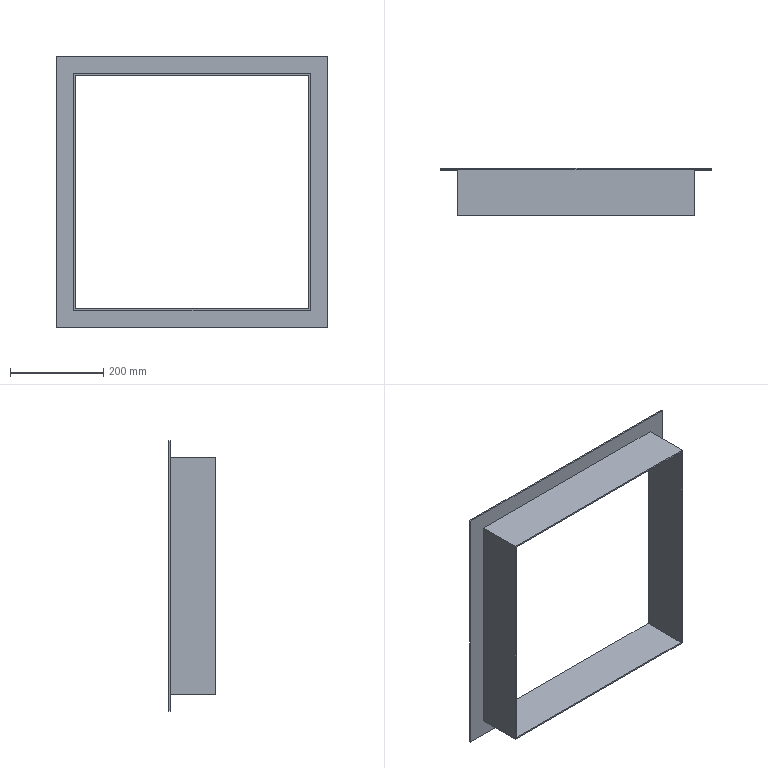Component | SolidWorks | Riser-1 | 1 solid | 15 faces | box 580 x 100 x 580 mm | volume 844692 mm3 | plane 15
build123d program:
from build123d import *


with BuildPart() as part:
    # Sweep1: sweep along a path in Sketch2
    with BuildLine(Plane(origin=(0, 0, 0), x_dir=(1, 0, 0), z_dir=(0, 1, 0))) as sweep1_path:
        Line((110.614, 658.612), (610.614, 658.612))
        Line((610.614, 658.612), (610.614, 158.612))
        Line((610.614, 158.612), (110.614, 158.612))
        Line((110.614, 158.612), (110.614, 658.612))
    # Sketch3 → Sweep1 (sweep)
    with BuildSketch(Plane.XY.offset(-158.612)):
        Polygon((610.614, 0), (610.614, 100), (650.614, 100), (650.614, 97), (613.614, 97), (613.614, 0), align=None)
    sweep(path=sweep1_path.line, transition=Transition.RIGHT)


solid = part.part

# Placed as in the assembly
solid = solid.moved(Location((520.859, 2190.46, 895.719), (0, 0, 0)))
STEP:
#1=CARTESIAN_POINT('',(44.546,86.239,29.02));
#2=VERTEX_POINT('',#1);
#3=CARTESIAN_POINT('',(44.546,90.176,29.02));
#4=VERTEX_POINT('',#3);
#5=CARTESIAN_POINT('',(44.546,86.239,29.02));
#6=CARTESIAN_POINT('',(44.546,87.551,29.02));
#7=CARTESIAN_POINT('',(44.546,88.863,29.02));
#8=CARTESIAN_POINT('',(44.546,90.176,29.02));
#9=B_SPLINE_CURVE_WITH_KNOTS('',3,(#5,#6,#7,#8),.UNSPECIFIED.,.F.,.F.,(4,4),(0.,1.),.UNSPECIFIED.);
#10=EDGE_CURVE('',#2,#4,#9,.T.);
#11=ORIENTED_EDGE('',*,*,#10,.F.);
#12=CARTESIAN_POINT('',(24.861,86.239,29.02));
#13=VERTEX_POINT('',#12);
#14=CARTESIAN_POINT('',(24.861,86.239,29.02));
#15=DIRECTION('',(1.,0.,0.));
#16=VECTOR('',#15,39.37);
#17=LINE('',#14,#16);
#18=EDGE_CURVE('',#13,#2,#17,.T.);
#19=ORIENTED_EDGE('',*,*,#18,.F.);
#20=CARTESIAN_POINT('',(24.861,90.176,29.02));
#21=VERTEX_POINT('',#20);
#22=CARTESIAN_POINT('',(24.861,86.239,29.02));
#23=DIRECTION('',(0.,-1.,0.));
#24=VECTOR('',#23,39.37);
#25=LINE('',#22,#24);
#26=EDGE_CURVE('',#21,#13,#25,.T.);
#27=ORIENTED_EDGE('',*,*,#26,.F.);
#28=CARTESIAN_POINT('',(24.861,90.176,29.02));
#29=DIRECTION('',(1.,0.,0.));
#30=VECTOR('',#29,39.37);
#31=LINE('',#28,#30);
#32=EDGE_CURVE('',#21,#4,#31,.T.);
#33=ORIENTED_EDGE('',*,*,#32,.T.);
#34=EDGE_LOOP('',(#11,#19,#27,#33));
#35=FACE_OUTER_BOUND('',#34,.T.);
#36=CARTESIAN_POINT('',(24.861,86.239,29.02));
#37=DIRECTION('',(0.,0.,1.));
#38=DIRECTION('',(1.,0.,0.));
#39=AXIS2_PLACEMENT_3D('',#36,#37,#38);
#40=PLANE('',#39);
#41=ADVANCED_FACE('',(#35),#40,.F.);
#42=CARTESIAN_POINT('',(44.664,90.057,29.138));
#43=VERTEX_POINT('',#42);
#44=CARTESIAN_POINT('',(44.664,86.239,29.138));
#45=VERTEX_POINT('',#44);
#46=CARTESIAN_POINT('',(44.664,90.057,29.138));
#47=CARTESIAN_POINT('',(44.664,88.785,29.138));
#48=CARTESIAN_POINT('',(44.664,87.512,29.138));
#49=CARTESIAN_POINT('',(44.664,86.239,29.138));
#50=B_SPLINE_CURVE_WITH_KNOTS('',3,(#46,#47,#48,#49),.UNSPECIFIED.,.F.,.F.,(4,4),(0.,1.),.UNSPECIFIED.);
#51=EDGE_CURVE('',#43,#45,#50,.T.);
#52=ORIENTED_EDGE('',*,*,#51,.F.);
#53=CARTESIAN_POINT('',(24.743,90.057,29.138));
#54=VERTEX_POINT('',#53);
#55=CARTESIAN_POINT('',(24.743,90.057,29.138));
#56=DIRECTION('',(1.,0.,0.));
#57=VECTOR('',#56,39.37);
#58=LINE('',#55,#57);
#59=EDGE_CURVE('',#54,#43,#58,.T.);
#60=ORIENTED_EDGE('',*,*,#59,.F.);
#61=CARTESIAN_POINT('',(24.743,86.239,29.138));
#62=VERTEX_POINT('',#61);
#63=CARTESIAN_POINT('',(24.743,90.057,29.138));
#64=DIRECTION('',(0.,1.,0.));
#65=VECTOR('',#64,39.37);
#66=LINE('',#63,#65);
#67=EDGE_CURVE('',#62,#54,#66,.T.);
#68=ORIENTED_EDGE('',*,*,#67,.F.);
#69=CARTESIAN_POINT('',(24.743,86.239,29.138));
#70=DIRECTION('',(1.,0.,0.));
#71=VECTOR('',#70,39.37);
#72=LINE('',#69,#71);
#73=EDGE_CURVE('',#62,#45,#72,.T.);
#74=ORIENTED_EDGE('',*,*,#73,.T.);
#75=EDGE_LOOP('',(#52,#60,#68,#74));
#76=FACE_OUTER_BOUND('',#75,.T.);
#77=CARTESIAN_POINT('',(24.743,90.057,29.138));
#78=DIRECTION('',(0.,0.,-1.));
#79=DIRECTION('',(-1.,0.,0.));
#80=AXIS2_PLACEMENT_3D('',#77,#78,#79);
#81=PLANE('',#80);
#82=ADVANCED_FACE('',(#76),#81,.F.);
#83=CARTESIAN_POINT('',(46.121,90.176,30.595));
#84=VERTEX_POINT('',#83);
#85=CARTESIAN_POINT('',(46.121,90.057,30.595));
#86=VERTEX_POINT('',#85);
#87=CARTESIAN_POINT('',(46.121,90.176,30.595));
#88=CARTESIAN_POINT('',(46.121,90.136,30.595));
#89=CARTESIAN_POINT('',(46.121,90.097,30.595));
#90=CARTESIAN_POINT('',(46.121,90.057,30.595));
#91=B_SPLINE_CURVE_WITH_KNOTS('',3,(#87,#88,#89,#90),.UNSPECIFIED.,.F.,.F.,(4,4),(0.,1.),.UNSPECIFIED.);
#92=EDGE_CURVE('',#84,#86,#91,.T.);
#93=ORIENTED_EDGE('',*,*,#92,.F.);
#94=CARTESIAN_POINT('',(23.286,90.176,30.595));
#95=VERTEX_POINT('',#94);
#96=CARTESIAN_POINT('',(23.286,90.176,30.595));
#97=DIRECTION('',(1.,0.,0.));
#98=VECTOR('',#97,39.37);
#99=LINE('',#96,#98);
#100=EDGE_CURVE('',#95,#84,#99,.T.);
#101=ORIENTED_EDGE('',*,*,#100,.F.);
#102=CARTESIAN_POINT('',(23.286,90.057,30.595));
#103=VERTEX_POINT('',#102);
#104=CARTESIAN_POINT('',(23.286,90.176,30.595));
#105=DIRECTION('',(0.,1.,0.));
#106=VECTOR('',#105,39.37);
#107=LINE('',#104,#106);
#108=EDGE_CURVE('',#103,#95,#107,.T.);
#109=ORIENTED_EDGE('',*,*,#108,.F.);
#110=CARTESIAN_POINT('',(23.286,90.057,30.595));
#111=DIRECTION('',(1.,0.,0.));
#112=VECTOR('',#111,39.37);
#113=LINE('',#110,#112);
#114=EDGE_CURVE('',#103,#86,#113,.T.);
#115=ORIENTED_EDGE('',*,*,#114,.T.);
#116=EDGE_LOOP('',(#93,#101,#109,#115));
#117=FACE_OUTER_BOUND('',#116,.T.);
#118=CARTESIAN_POINT('',(23.286,90.176,30.595));
#119=DIRECTION('',(0.,0.,-1.));
#120=DIRECTION('',(-1.,0.,0.));
#121=AXIS2_PLACEMENT_3D('',#118,#119,#120);
#122=PLANE('',#121);
#123=ADVANCED_FACE('',(#117),#122,.F.);
#124=CARTESIAN_POINT('',(24.861,90.176,9.335));
#125=VERTEX_POINT('',#124);
#126=CARTESIAN_POINT('',(24.861,90.176,9.335));
#127=DIRECTION('',(0.,0.,1.));
#128=VECTOR('',#127,39.37);
#129=LINE('',#126,#128);
#130=EDGE_CURVE('',#125,#21,#129,.T.);
#131=ORIENTED_EDGE('',*,*,#130,.T.);
#132=ORIENTED_EDGE('',*,*,#26,.T.);
#133=CARTESIAN_POINT('',(24.861,86.239,9.335));
#134=VERTEX_POINT('',#133);
#135=CARTESIAN_POINT('',(24.861,86.239,9.335));
#136=DIRECTION('',(0.,0.,1.));
#137=VECTOR('',#136,39.37);
#138=LINE('',#135,#137);
#139=EDGE_CURVE('',#134,#13,#138,.T.);
#140=ORIENTED_EDGE('',*,*,#139,.F.);
#141=CARTESIAN_POINT('',(24.861,86.239,9.335));
#142=DIRECTION('',(0.,1.,0.));
#143=VECTOR('',#142,39.37);
#144=LINE('',#141,#143);
#145=EDGE_CURVE('',#134,#125,#144,.T.);
#146=ORIENTED_EDGE('',*,*,#145,.T.);
#147=EDGE_LOOP('',(#131,#132,#140,#146));
#148=FACE_OUTER_BOUND('',#147,.T.);
#149=CARTESIAN_POINT('',(24.861,86.239,9.335));
#150=DIRECTION('',(1.,0.,-0.));
#151=DIRECTION('',(-0.,0.,-1.));
#152=AXIS2_PLACEMENT_3D('',#149,#150,#151);
#153=PLANE('',#152);
#154=ADVANCED_FACE('',(#148),#153,.T.);
#155=CARTESIAN_POINT('',(24.743,86.239,9.217));
#156=VERTEX_POINT('',#155);
#157=CARTESIAN_POINT('',(24.743,86.239,9.217));
#158=DIRECTION('',(0.,0.,1.));
#159=VECTOR('',#158,39.37);
#160=LINE('',#157,#159);
#161=EDGE_CURVE('',#156,#62,#160,.T.);
#162=ORIENTED_EDGE('',*,*,#161,.T.);
#163=ORIENTED_EDGE('',*,*,#67,.T.);
#164=CARTESIAN_POINT('',(24.743,90.057,9.217));
#165=VERTEX_POINT('',#164);
#166=CARTESIAN_POINT('',(24.743,90.057,9.217));
#167=DIRECTION('',(0.,0.,1.));
#168=VECTOR('',#167,39.37);
#169=LINE('',#166,#168);
#170=EDGE_CURVE('',#165,#54,#169,.T.);
#171=ORIENTED_EDGE('',*,*,#170,.F.);
#172=CARTESIAN_POINT('',(24.743,90.057,9.217));
#173=DIRECTION('',(0.,-1.,0.));
#174=VECTOR('',#173,39.37);
#175=LINE('',#172,#174);
#176=EDGE_CURVE('',#165,#156,#175,.T.);
#177=ORIENTED_EDGE('',*,*,#176,.T.);
#178=EDGE_LOOP('',(#162,#163,#171,#177));
#179=FACE_OUTER_BOUND('',#178,.T.);
#180=CARTESIAN_POINT('',(24.743,90.057,9.217));
#181=DIRECTION('',(-1.,0.,0.));
#182=DIRECTION('',(0.,0.,1.));
#183=AXIS2_PLACEMENT_3D('',#180,#181,#182);
#184=PLANE('',#183);
#185=ADVANCED_FACE('',(#179),#184,.T.);
#186=CARTESIAN_POINT('',(23.286,90.057,7.76));
#187=VERTEX_POINT('',#186);
#188=CARTESIAN_POINT('',(23.286,90.057,7.76));
#189=DIRECTION('',(0.,0.,1.));
#190=VECTOR('',#189,39.37);
#191=LINE('',#188,#190);
#192=EDGE_CURVE('',#187,#103,#191,.T.);
#193=ORIENTED_EDGE('',*,*,#192,.T.);
#194=ORIENTED_EDGE('',*,*,#108,.T.);
#195=CARTESIAN_POINT('',(23.286,90.176,7.76));
#196=VERTEX_POINT('',#195);
#197=CARTESIAN_POINT('',(23.286,90.176,7.76));
#198=DIRECTION('',(0.,0.,1.));
#199=VECTOR('',#198,39.37);
#200=LINE('',#197,#199);
#201=EDGE_CURVE('',#196,#95,#200,.T.);
#202=ORIENTED_EDGE('',*,*,#201,.F.);
#203=CARTESIAN_POINT('',(23.286,90.176,7.76));
#204=DIRECTION('',(0.,-1.,0.));
#205=VECTOR('',#204,39.37);
#206=LINE('',#203,#205);
#207=EDGE_CURVE('',#196,#187,#206,.T.);
#208=ORIENTED_EDGE('',*,*,#207,.T.);
#209=EDGE_LOOP('',(#193,#194,#202,#208));
#210=FACE_OUTER_BOUND('',#209,.T.);
#211=CARTESIAN_POINT('',(23.286,90.176,7.76));
#212=DIRECTION('',(-1.,0.,0.));
#213=DIRECTION('',(0.,0.,1.));
#214=AXIS2_PLACEMENT_3D('',#211,#212,#213);
#215=PLANE('',#214);
#216=ADVANCED_FACE('',(#210),#215,.T.);
#217=ORIENTED_EDGE('',*,*,#145,.F.);
#218=CARTESIAN_POINT('',(44.546,86.239,9.335));
#219=VERTEX_POINT('',#218);
#220=CARTESIAN_POINT('',(44.546,86.239,9.335));
#221=DIRECTION('',(-1.,0.,0.));
#222=VECTOR('',#221,39.37);
#223=LINE('',#220,#222);
#224=EDGE_CURVE('',#219,#134,#223,.T.);
#225=ORIENTED_EDGE('',*,*,#224,.F.);
#226=CARTESIAN_POINT('',(44.546,90.176,9.335));
#227=VERTEX_POINT('',#226);
#228=CARTESIAN_POINT('',(44.546,86.239,9.335));
#229=DIRECTION('',(0.,-1.,0.));
#230=VECTOR('',#229,39.37);
#231=LINE('',#228,#230);
#232=EDGE_CURVE('',#227,#219,#231,.T.);
#233=ORIENTED_EDGE('',*,*,#232,.F.);
#234=CARTESIAN_POINT('',(44.546,90.176,9.335));
#235=DIRECTION('',(-1.,0.,0.));
#236=VECTOR('',#235,39.37);
#237=LINE('',#234,#236);
#238=EDGE_CURVE('',#227,#125,#237,.T.);
#239=ORIENTED_EDGE('',*,*,#238,.T.);
#240=EDGE_LOOP('',(#217,#225,#233,#239));
#241=FACE_OUTER_BOUND('',#240,.T.);
#242=CARTESIAN_POINT('',(44.546,86.239,9.335));
#243=DIRECTION('',(0.,0.,-1.));
#244=DIRECTION('',(-1.,0.,0.));
#245=AXIS2_PLACEMENT_3D('',#242,#243,#244);
#246=PLANE('',#245);
#247=ADVANCED_FACE('',(#241),#246,.F.);
#248=ORIENTED_EDGE('',*,*,#176,.F.);
#249=CARTESIAN_POINT('',(44.664,90.057,9.217));
#250=VERTEX_POINT('',#249);
#251=CARTESIAN_POINT('',(44.664,90.057,9.217));
#252=DIRECTION('',(-1.,0.,0.));
#253=VECTOR('',#252,39.37);
#254=LINE('',#251,#253);
#255=EDGE_CURVE('',#250,#165,#254,.T.);
#256=ORIENTED_EDGE('',*,*,#255,.F.);
#257=CARTESIAN_POINT('',(44.664,86.239,9.217));
#258=VERTEX_POINT('',#257);
#259=CARTESIAN_POINT('',(44.664,90.057,9.217));
#260=DIRECTION('',(0.,1.,0.));
#261=VECTOR('',#260,39.37);
#262=LINE('',#259,#261);
#263=EDGE_CURVE('',#258,#250,#262,.T.);
#264=ORIENTED_EDGE('',*,*,#263,.F.);
#265=CARTESIAN_POINT('',(44.664,86.239,9.217));
#266=DIRECTION('',(-1.,0.,0.));
#267=VECTOR('',#266,39.37);
#268=LINE('',#265,#267);
#269=EDGE_CURVE('',#258,#156,#268,.T.);
#270=ORIENTED_EDGE('',*,*,#269,.T.);
#271=EDGE_LOOP('',(#248,#256,#264,#270));
#272=FACE_OUTER_BOUND('',#271,.T.);
#273=CARTESIAN_POINT('',(44.664,90.057,9.217));
#274=DIRECTION('',(0.,0.,1.));
#275=DIRECTION('',(1.,0.,0.));
#276=AXIS2_PLACEMENT_3D('',#273,#274,#275);
#277=PLANE('',#276);
#278=ADVANCED_FACE('',(#272),#277,.F.);
#279=ORIENTED_EDGE('',*,*,#207,.F.);
#280=CARTESIAN_POINT('',(46.121,90.176,7.76));
#281=VERTEX_POINT('',#280);
#282=CARTESIAN_POINT('',(46.121,90.176,7.76));
#283=DIRECTION('',(-1.,0.,0.));
#284=VECTOR('',#283,39.37);
#285=LINE('',#282,#284);
#286=EDGE_CURVE('',#281,#196,#285,.T.);
#287=ORIENTED_EDGE('',*,*,#286,.F.);
#288=CARTESIAN_POINT('',(46.121,90.057,7.76));
#289=VERTEX_POINT('',#288);
#290=CARTESIAN_POINT('',(46.121,90.176,7.76));
#291=DIRECTION('',(0.,1.,0.));
#292=VECTOR('',#291,39.37);
#293=LINE('',#290,#292);
#294=EDGE_CURVE('',#289,#281,#293,.T.);
#295=ORIENTED_EDGE('',*,*,#294,.F.);
#296=CARTESIAN_POINT('',(46.121,90.057,7.76));
#297=DIRECTION('',(-1.,0.,0.));
#298=VECTOR('',#297,39.37);
#299=LINE('',#296,#298);
#300=EDGE_CURVE('',#289,#187,#299,.T.);
#301=ORIENTED_EDGE('',*,*,#300,.T.);
#302=EDGE_LOOP('',(#279,#287,#295,#301));
#303=FACE_OUTER_BOUND('',#302,.T.);
#304=CARTESIAN_POINT('',(46.121,90.176,7.76));
#305=DIRECTION('',(0.,0.,1.));
#306=DIRECTION('',(1.,0.,0.));
#307=AXIS2_PLACEMENT_3D('',#304,#305,#306);
#308=PLANE('',#307);
#309=ADVANCED_FACE('',(#303),#308,.F.);
#310=CARTESIAN_POINT('',(44.664,86.239,-0.7204));
#311=DIRECTION('',(0.,0.,1.));
#312=VECTOR('',#311,39.37);
#313=LINE('',#310,#312);
#314=EDGE_CURVE('',#258,#45,#313,.T.);
#315=ORIENTED_EDGE('',*,*,#314,.F.);
#316=ORIENTED_EDGE('',*,*,#263,.T.);
#317=CARTESIAN_POINT('',(44.664,90.057,-0.7204));
#318=DIRECTION('',(0.,0.,1.));
#319=VECTOR('',#318,39.37);
#320=LINE('',#317,#319);
#321=EDGE_CURVE('',#250,#43,#320,.T.);
#322=ORIENTED_EDGE('',*,*,#321,.T.);
#323=ORIENTED_EDGE('',*,*,#51,.T.);
#324=EDGE_LOOP('',(#315,#316,#322,#323));
#325=FACE_OUTER_BOUND('',#324,.T.);
#326=CARTESIAN_POINT('',(44.664,90.057,-0.7204));
#327=DIRECTION('',(1.,0.,-0.));
#328=DIRECTION('',(-0.,0.,-1.));
#329=AXIS2_PLACEMENT_3D('',#326,#327,#328);
#330=PLANE('',#329);
#331=ADVANCED_FACE('',(#325),#330,.T.);
#332=ORIENTED_EDGE('',*,*,#300,.F.);
#333=CARTESIAN_POINT('',(46.121,90.057,-0.7204));
#334=DIRECTION('',(0.,0.,1.));
#335=VECTOR('',#334,39.37);
#336=LINE('',#333,#335);
#337=EDGE_CURVE('',#289,#86,#336,.T.);
#338=ORIENTED_EDGE('',*,*,#337,.T.);
#339=ORIENTED_EDGE('',*,*,#114,.F.);
#340=ORIENTED_EDGE('',*,*,#192,.F.);
#341=EDGE_LOOP('',(#332,#338,#339,#340));
#342=FACE_OUTER_BOUND('',#341,.T.);
#343=ORIENTED_EDGE('',*,*,#321,.F.);
#344=ORIENTED_EDGE('',*,*,#255,.T.);
#345=ORIENTED_EDGE('',*,*,#170,.T.);
#346=ORIENTED_EDGE('',*,*,#59,.T.);
#347=EDGE_LOOP('',(#343,#344,#345,#346));
#348=FACE_BOUND('',#347,.T.);
#349=CARTESIAN_POINT('',(46.121,90.057,-0.7204));
#350=DIRECTION('',(0.,-1.,0.));
#351=DIRECTION('',(0.,0.,-1.));
#352=AXIS2_PLACEMENT_3D('',#349,#350,#351);
#353=PLANE('',#352);
#354=ADVANCED_FACE('',(#342,#348),#353,.T.);
#355=ORIENTED_EDGE('',*,*,#337,.F.);
#356=ORIENTED_EDGE('',*,*,#294,.T.);
#357=CARTESIAN_POINT('',(46.121,90.176,-0.7204));
#358=DIRECTION('',(0.,0.,1.));
#359=VECTOR('',#358,39.37);
#360=LINE('',#357,#359);
#361=EDGE_CURVE('',#281,#84,#360,.T.);
#362=ORIENTED_EDGE('',*,*,#361,.T.);
#363=ORIENTED_EDGE('',*,*,#92,.T.);
#364=EDGE_LOOP('',(#355,#356,#362,#363));
#365=FACE_OUTER_BOUND('',#364,.T.);
#366=CARTESIAN_POINT('',(46.121,90.176,-0.7204));
#367=DIRECTION('',(1.,0.,-0.));
#368=DIRECTION('',(-0.,0.,-1.));
#369=AXIS2_PLACEMENT_3D('',#366,#367,#368);
#370=PLANE('',#369);
#371=ADVANCED_FACE('',(#365),#370,.T.);
#372=ORIENTED_EDGE('',*,*,#238,.F.);
#373=CARTESIAN_POINT('',(44.546,90.176,-0.7204));
#374=DIRECTION('',(0.,0.,1.));
#375=VECTOR('',#374,39.37);
#376=LINE('',#373,#375);
#377=EDGE_CURVE('',#227,#4,#376,.T.);
#378=ORIENTED_EDGE('',*,*,#377,.T.);
#379=ORIENTED_EDGE('',*,*,#32,.F.);
#380=ORIENTED_EDGE('',*,*,#130,.F.);
#381=EDGE_LOOP('',(#372,#378,#379,#380));
#382=FACE_BOUND('',#381,.T.);
#383=ORIENTED_EDGE('',*,*,#361,.F.);
#384=ORIENTED_EDGE('',*,*,#286,.T.);
#385=ORIENTED_EDGE('',*,*,#201,.T.);
#386=ORIENTED_EDGE('',*,*,#100,.T.);
#387=EDGE_LOOP('',(#383,#384,#385,#386));
#388=FACE_OUTER_BOUND('',#387,.T.);
#389=CARTESIAN_POINT('',(44.546,90.176,-0.7204));
#390=DIRECTION('',(0.,1.,0.));
#391=DIRECTION('',(0.,0.,1.));
#392=AXIS2_PLACEMENT_3D('',#389,#390,#391);
#393=PLANE('',#392);
#394=ADVANCED_FACE('',(#382,#388),#393,.T.);
#395=ORIENTED_EDGE('',*,*,#377,.F.);
#396=ORIENTED_EDGE('',*,*,#232,.T.);
#397=CARTESIAN_POINT('',(44.546,86.239,-0.7204));
#398=DIRECTION('',(0.,0.,1.));
#399=VECTOR('',#398,39.37);
#400=LINE('',#397,#399);
#401=EDGE_CURVE('',#219,#2,#400,.T.);
#402=ORIENTED_EDGE('',*,*,#401,.T.);
#403=ORIENTED_EDGE('',*,*,#10,.T.);
#404=EDGE_LOOP('',(#395,#396,#402,#403));
#405=FACE_OUTER_BOUND('',#404,.T.);
#406=CARTESIAN_POINT('',(44.546,86.239,-0.7204));
#407=DIRECTION('',(-1.,0.,0.));
#408=DIRECTION('',(0.,0.,1.));
#409=AXIS2_PLACEMENT_3D('',#406,#407,#408);
#410=PLANE('',#409);
#411=ADVANCED_FACE('',(#405),#410,.T.);
#412=ORIENTED_EDGE('',*,*,#269,.F.);
#413=ORIENTED_EDGE('',*,*,#314,.T.);
#414=ORIENTED_EDGE('',*,*,#73,.F.);
#415=ORIENTED_EDGE('',*,*,#161,.F.);
#416=EDGE_LOOP('',(#412,#413,#414,#415));
#417=FACE_OUTER_BOUND('',#416,.T.);
#418=ORIENTED_EDGE('',*,*,#401,.F.);
#419=ORIENTED_EDGE('',*,*,#224,.T.);
#420=ORIENTED_EDGE('',*,*,#139,.T.);
#421=ORIENTED_EDGE('',*,*,#18,.T.);
#422=EDGE_LOOP('',(#418,#419,#420,#421));
#423=FACE_BOUND('',#422,.T.);
#424=CARTESIAN_POINT('',(44.664,86.239,-0.7204));
#425=DIRECTION('',(-0.,-1.,0.));
#426=DIRECTION('',(1.,-0.,0.));
#427=AXIS2_PLACEMENT_3D('',#424,#425,#426);
#428=PLANE('',#427);
#429=ADVANCED_FACE('',(#417,#423),#428,.T.);
#430=CLOSED_SHELL('',(#41,#82,#123,#154,#185,#216,#247,#278,#309,#331,#354,#371,#394,#411,#429));
#431=MANIFOLD_SOLID_BREP('',#430);
#432=CARTESIAN_POINT('',(0.,0.,0.));
#433=DIRECTION('',(0.,0.,1.));
#434=DIRECTION('',(1.,0.,0.));
#435=AXIS2_PLACEMENT_3D('',#432,#433,#434);
#436=(LENGTH_UNIT()NAMED_UNIT(*)SI_UNIT($,.METRE.));
#437=LENGTH_MEASURE_WITH_UNIT(LENGTH_MEASURE(0.0254),#436);
#438=DIMENSIONAL_EXPONENTS(1.,0.,0.,0.,0.,0.,0.);
#439=(CONVERSION_BASED_UNIT('',#437)LENGTH_UNIT()NAMED_UNIT(#438));
#440=UNCERTAINTY_MEASURE_WITH_UNIT(LENGTH_MEASURE(0.00001),#439,'','');
#441=(NAMED_UNIT(*)PLANE_ANGLE_UNIT()SI_UNIT($,.RADIAN.));
#442=(NAMED_UNIT(*)SI_UNIT($,.STERADIAN.)SOLID_ANGLE_UNIT());
#443=(GEOMETRIC_REPRESENTATION_CONTEXT(3)GLOBAL_UNCERTAINTY_ASSIGNED_CONTEXT((#440))GLOBAL_UNIT_ASSIGNED_CONTEXT((#439,#441,#442))REPRESENTATION_CONTEXT('',''));
#444=ADVANCED_BREP_SHAPE_REPRESENTATION('',(#431,#435),#443);
#445=COLOUR_RGB('',0.7922,0.8196,0.9333);
#446=FILL_AREA_STYLE_COLOUR('',#445);
#447=FILL_AREA_STYLE('',(#446));
#448=SURFACE_STYLE_FILL_AREA(#447);
#449=SURFACE_SIDE_STYLE('',(#448));
#450=SURFACE_STYLE_USAGE(.BOTH.,#449);
#451=PRESENTATION_STYLE_ASSIGNMENT((#450));
#452=STYLED_ITEM('',(#451),#431);
#453=(LENGTH_UNIT()NAMED_UNIT(*)SI_UNIT($,.METRE.));
#454=LENGTH_MEASURE_WITH_UNIT(LENGTH_MEASURE(0.0254),#453);
#455=DIMENSIONAL_EXPONENTS(1.,0.,0.,0.,0.,0.,0.);
#456=(CONVERSION_BASED_UNIT('',#454)LENGTH_UNIT()NAMED_UNIT(#455));
#457=UNCERTAINTY_MEASURE_WITH_UNIT(LENGTH_MEASURE(0.00001),#456,'','');
#458=(NAMED_UNIT(*)PLANE_ANGLE_UNIT()SI_UNIT($,.RADIAN.));
#459=(NAMED_UNIT(*)SI_UNIT($,.STERADIAN.)SOLID_ANGLE_UNIT());
#460=(GEOMETRIC_REPRESENTATION_CONTEXT(3)GLOBAL_UNCERTAINTY_ASSIGNED_CONTEXT((#457))GLOBAL_UNIT_ASSIGNED_CONTEXT((#456,#458,#459))REPRESENTATION_CONTEXT('',''));
#461=MECHANICAL_DESIGN_GEOMETRIC_PRESENTATION_REPRESENTATION('',(#452),#460);
#462=PRESENTATION_LAYER_ASSIGNMENT('','',(#452));